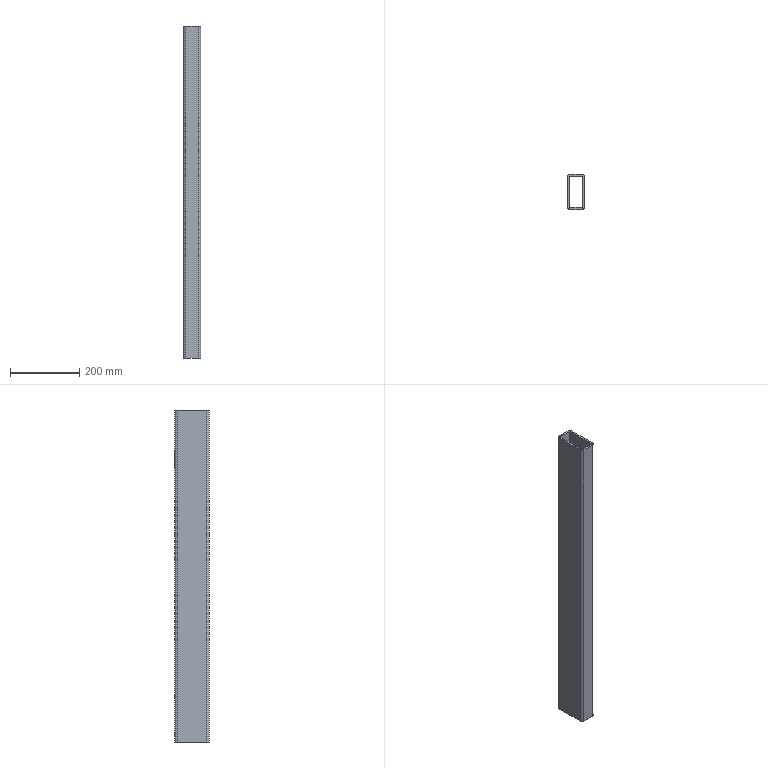Component | SolidWorks | JHK-A1004LeftRectangularTubeBeam-1 | 1 solid | 42 faces | box 50 x 100 x 960 mm | volume 1271921 mm3 | cylinder 24 | plane 18 | commonest cylinder face diameters 5 x8 15 x4 20 x4 10 x4 6.8 x2 30 x2 | material Q235A
build123d program:
from build123d import *

# Parameters (mm, degrees)
EXTRUDE_THIN1_DEPTH   = 480
CUT_EXTRUDE1_REACH    = 487.18
SKETCH2_R             = 15
CUT_EXTRUDE2_REACH    = 487.18
CUT_EXTRUDE4_REACH    = 492.943
M6_TAPPED_HOLE1_D     = 5
M6_TAPPED_HOLE1_DEPTH = 5
M8_TAPPED_HOLE1_D     = 6.8
M8_TAPPED_HOLE1_DEPTH = 5


with BuildPart() as part:
    # Sketch1 → Extrude-Thin1 (new, symmetric)
    with BuildSketch(Plane.XY):
        with BuildLine():
            Line((17.5, 50), (-17.5, 50))
            ThreePointArc((-17.5, 50), (-22.803, 47.803), (-25, 42.5))
            Line((-25, 42.5), (-25, -42.5))
            ThreePointArc((-25, -42.5), (-22.803, -47.803), (-17.5, -50))
            Line((-17.5, -50), (17.5, -50))
            ThreePointArc((17.5, -50), (22.803, -47.803), (25, -42.5))
            Line((25, -42.5), (25, 42.5))
            ThreePointArc((25, 42.5), (22.803, 47.803), (17.5, 50))
        make_face()
        with BuildLine():
            Line((17.5, 45), (-17.5, 45))
            ThreePointArc((-17.5, 45), (-19.268, 44.268), (-20, 42.5))
            Line((-20, 42.5), (-20, -42.5))
            ThreePointArc((-20, -42.5), (-19.268, -44.268), (-17.5, -45))
            Line((-17.5, -45), (17.5, -45))
            ThreePointArc((17.5, -45), (19.268, -44.268), (20, -42.5))
            Line((20, -42.5), (20, 42.5))
            ThreePointArc((20, 42.5), (19.268, 44.268), (17.5, 45))
        make_face(mode=Mode.SUBTRACT)
    extrude(amount=EXTRUDE_THIN1_DEPTH, both=True)

    # Sketch2 → Cut-Extrude1 (cut, up to next)
    with BuildSketch(Plane.ZY.offset(-25), mode=Mode.PRIVATE) as cut_extrude1_sk1:
        with Locations((-430, 0)):
            Circle(SKETCH2_R)
    cut_extrude1_tool1 = extrude(cut_extrude1_sk1.sketch, amount=CUT_EXTRUDE1_REACH, mode=Mode.PRIVATE) & part.part
    add(cut_extrude1_tool1.solids().sort_by_distance((25, 0, -430))[0], mode=Mode.SUBTRACT)

    # Sketch5 → Cut-Extrude2 (cut, up to next)
    with BuildSketch(Plane(origin=(25, 0, 0), x_dir=(0, 0, -1), z_dir=(1, 0, 0)), mode=Mode.PRIVATE) as cut_extrude2_sk1:
        with BuildLine():
            Line((200, -25), (270, -25))
            ThreePointArc((270, -25), (277.071, -22.071), (280, -15))
            Line((280, -15), (280, 15))
            ThreePointArc((280, 15), (277.071, 22.071), (270, 25))
            Line((270, 25), (200, 25))
            ThreePointArc((200, 25), (192.929, 22.071), (190, 15))
            Line((190, 15), (190, -15))
            ThreePointArc((190, -15), (192.929, -22.071), (200, -25))
        make_face()
    cut_extrude2_tool1 = extrude(cut_extrude2_sk1.sketch, amount=-CUT_EXTRUDE2_REACH, mode=Mode.PRIVATE) & part.part
    add(cut_extrude2_tool1.solids().sort_by_distance((25, 0, -235))[0], mode=Mode.SUBTRACT)

    # Sketch7 → Cut-Extrude4 (cut, up to next)
    with BuildSketch(Plane(origin=(0, 50, 0), x_dir=(1, 0, 0), z_dir=(0, 1, 0)), mode=Mode.PRIVATE) as cut_extrude4_sk1:
        with BuildLine():
            Line((-5, -360), (5, -360))
            ThreePointArc((5, -360), (8.536, -358.536), (10, -355))
            Line((10, -355), (10, -315))
            ThreePointArc((10, -315), (8.536, -311.464), (5, -310))
            Line((5, -310), (-5, -310))
            ThreePointArc((-5, -310), (-8.536, -311.464), (-10, -315))
            Line((-10, -315), (-10, -355))
            ThreePointArc((-10, -355), (-8.536, -358.536), (-5, -360))
        make_face()
    cut_extrude4_tool1 = extrude(cut_extrude4_sk1.sketch, amount=-CUT_EXTRUDE4_REACH, mode=Mode.PRIVATE) & part.part
    add(cut_extrude4_tool1.solids().sort_by_distance((0, 50, 335))[0], mode=Mode.SUBTRACT)

    # M6 Tapped Hole1
    with Locations(Plane(origin=(0, 50, 0), x_dir=(1, 0, 0), z_dir=(0, 1, 0))):
        with Locations((0, 457.5), (0, 347.5)):
            Hole(M6_TAPPED_HOLE1_D / 2, depth=M6_TAPPED_HOLE1_DEPTH)

    # M8 Tapped Hole1
    with Locations(Plane(origin=(0, 50, 0), x_dir=(1, 0, 0), z_dir=(0, 1, 0))):
        with Locations((0, -50)):
            Hole(M8_TAPPED_HOLE1_D / 2, depth=M8_TAPPED_HOLE1_DEPTH)


solid = part.part

# Placed as in the assembly
solid = solid.moved(Location((-155, -105, -761), (0, 0, 0)))